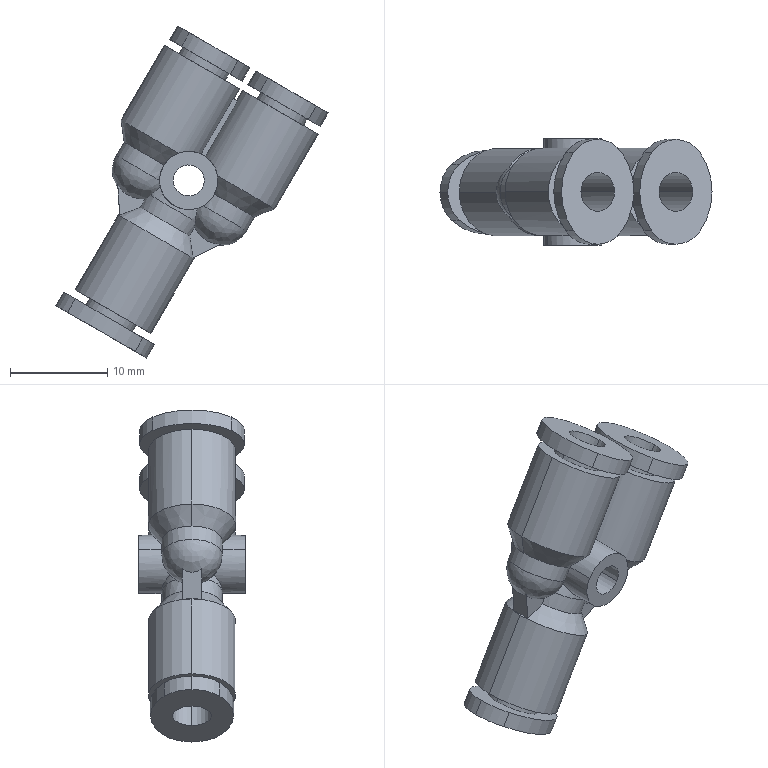Component | SolidWorks | Y-Joint-1 | 1 solid | 76 faces | volume 2262 mm3 | cylinder 44 | plane 23 | cone 5 | spline 4 | commonest cylinder face diameters 12.817 x8 7.4 x7 9 x6 5.5 x6 4 x6 6.2 x5 6 x4 3.2 x2